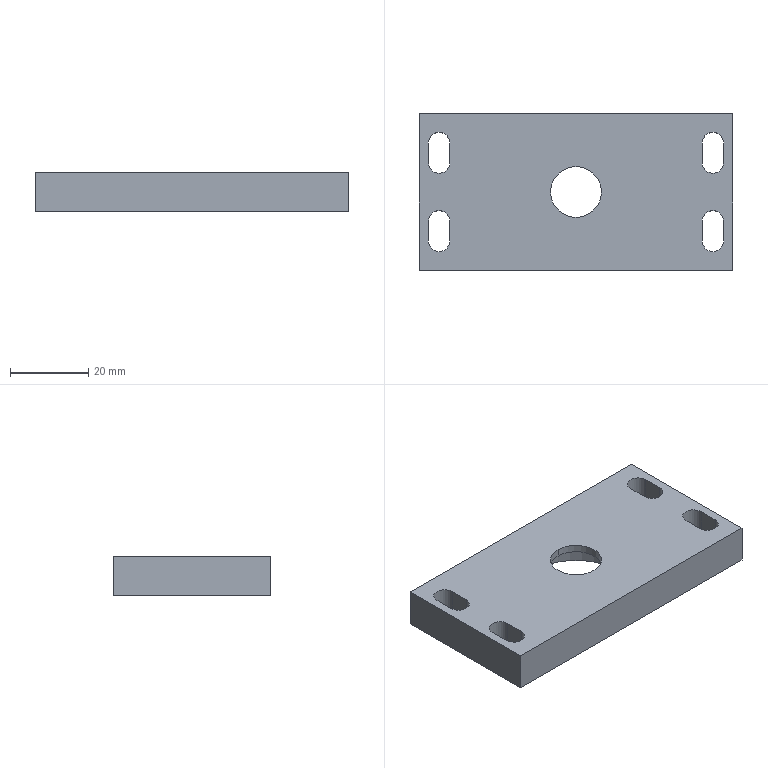CAM job | Mastercam | mm | 8 operations | part box 80 x 40 x 10
1. Contour (Ramp) | 1 - 8 平铣刀
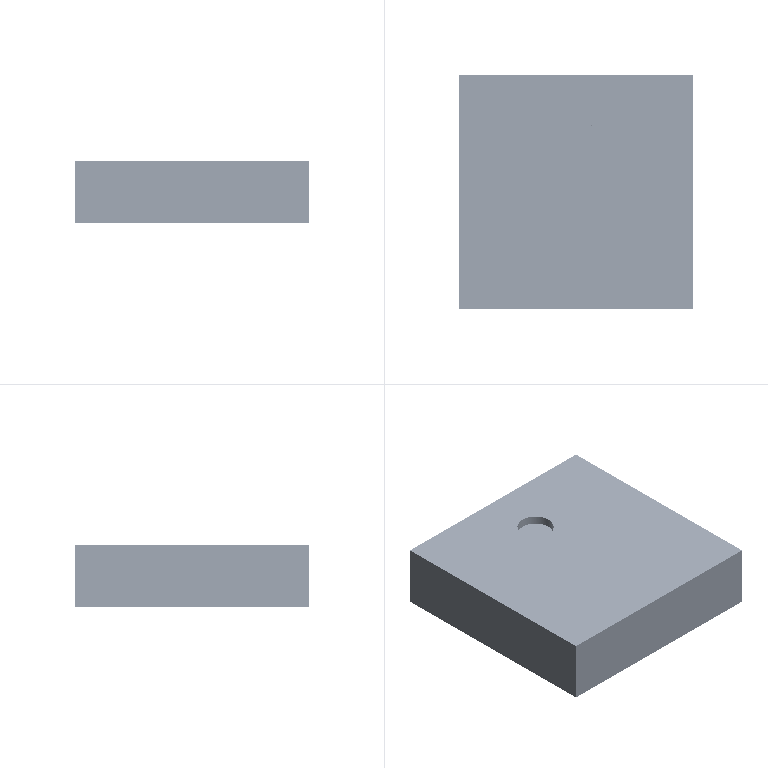2. Contour (2D) | 2 - 8 平铣刀
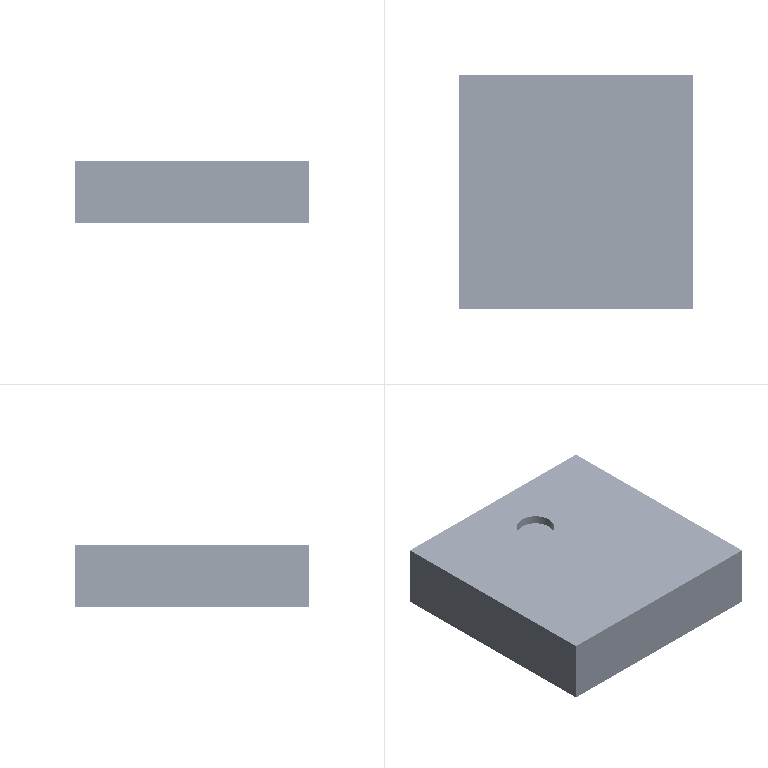3. Contour (Ramp) | 3 - 4 平铣刀
4. Contour (2D) | 4 - 4 平铣刀
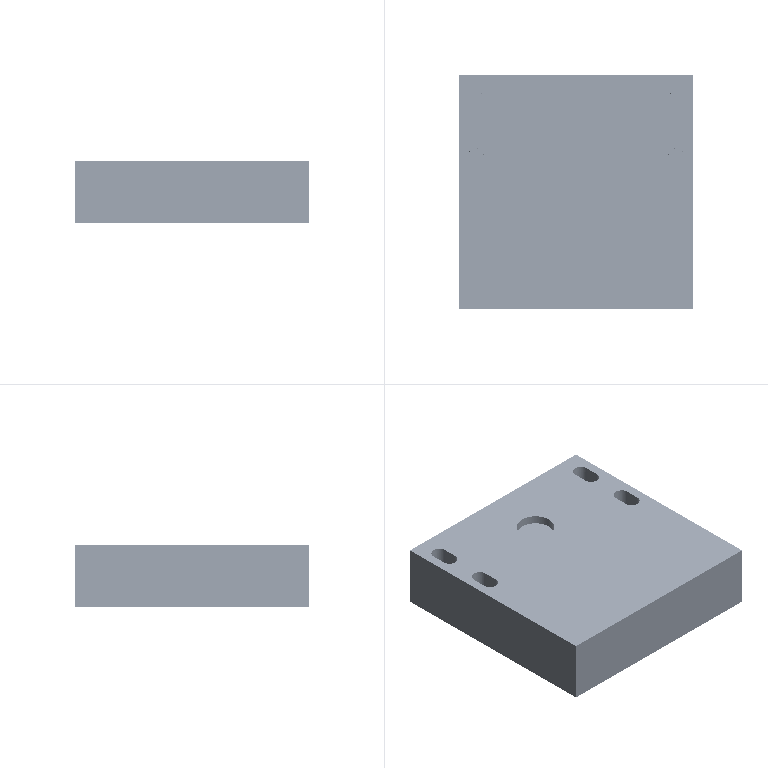5. Model Chamfer | 5 - 6 倒角刀
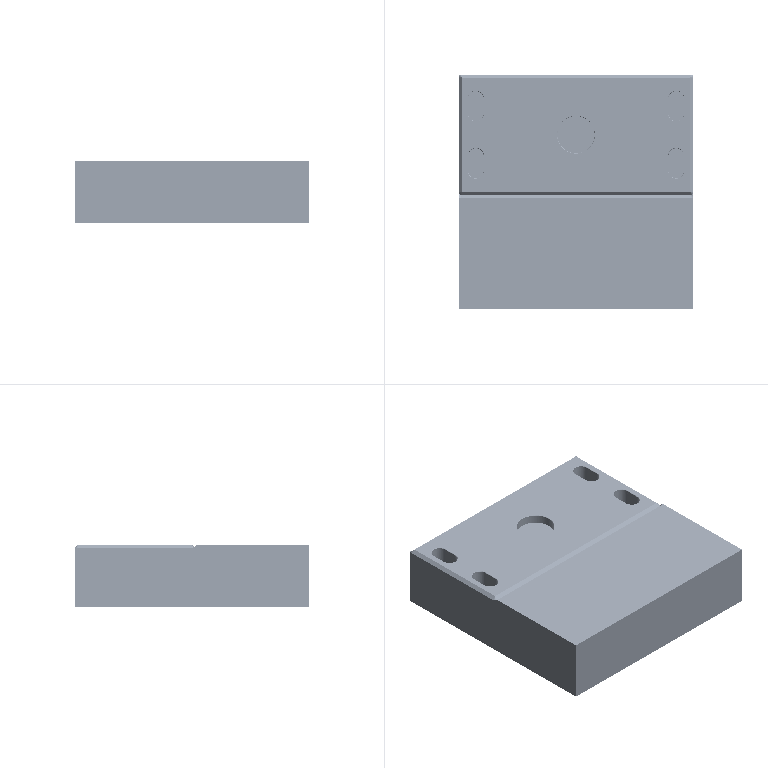6. Contour (Ramp) | 1 - 8 平铣刀
7. Contour (2D) | 2 - 8 平铣刀
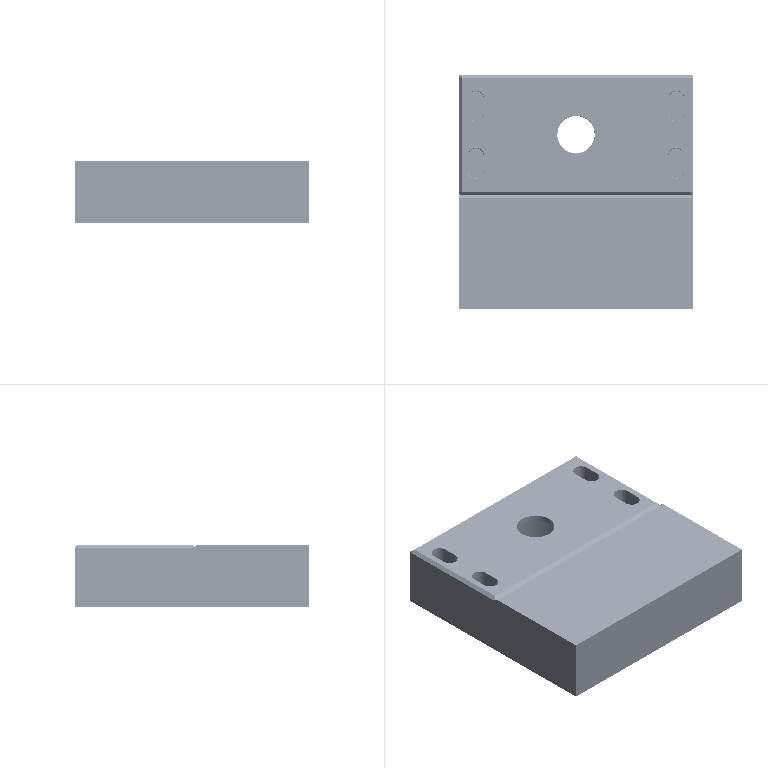8. Model Chamfer | 5 - 6 倒角刀